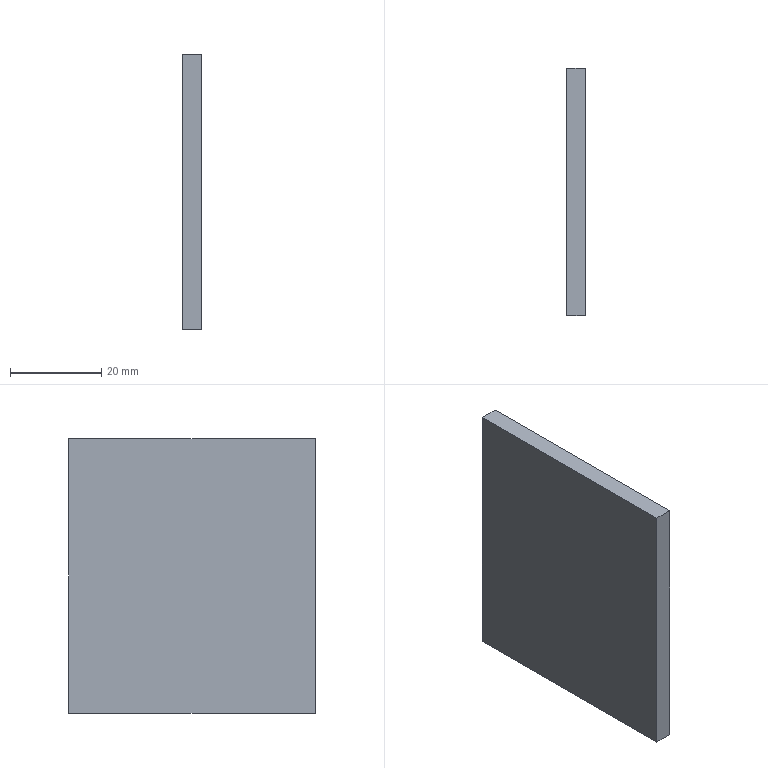Component | SolidWorks | RubberPlate-1 | 1 solid | 6 faces | box 4 x 54 x 60 mm | volume 12960 mm3 | plane 6
build123d program:
from build123d import *

# Parameters (mm, degrees)
SKETCH1_W           = 54
SKETCH1_H           = 60
BOSS_EXTRUDE1_DEPTH = 4


with BuildPart() as part:
    # Sketch1 → Boss-Extrude1 (new body)
    with BuildSketch(Plane(origin=(0, 0, -2), x_dir=(-1, 0, 0), z_dir=(0, 0, -1))):
        Rectangle(SKETCH1_W, SKETCH1_H)
    extrude(amount=-BOSS_EXTRUDE1_DEPTH)


solid = part.part

# Placed as in the assembly
solid = solid.moved(Location((-386, 405.75, -73.487), (90, -90, 0)))
STEP:
#1=COLOUR_RGB('',0.7922,0.8196,0.9333);
#2=FILL_AREA_STYLE_COLOUR('',#1);
#3=FILL_AREA_STYLE('',(#2));
#4=SURFACE_STYLE_FILL_AREA(#3);
#5=SURFACE_SIDE_STYLE('',(#4));
#6=SURFACE_STYLE_USAGE(.BOTH.,#5);
#7=PRESENTATION_STYLE_ASSIGNMENT((#6));
#8=CARTESIAN_POINT('',(-15.118,17.037,-1.712));
#9=VERTEX_POINT('',#8);
#10=CARTESIAN_POINT('',(-15.118,14.911,-1.712));
#11=VERTEX_POINT('',#10);
#12=CARTESIAN_POINT('',(-15.118,17.037,-1.712));
#13=DIRECTION('',(-0.,-1.,0.));
#14=VECTOR('',#13,39.37);
#15=LINE('',#12,#14);
#16=EDGE_CURVE('',#9,#11,#15,.T.);
#17=ORIENTED_EDGE('',*,*,#16,.F.);
#18=CARTESIAN_POINT('',(-15.276,17.037,-1.712));
#19=VERTEX_POINT('',#18);
#20=CARTESIAN_POINT('',(-15.276,17.037,-1.712));
#21=DIRECTION('',(1.,-0.,0.));
#22=VECTOR('',#21,39.37);
#23=LINE('',#20,#22);
#24=EDGE_CURVE('',#19,#9,#23,.T.);
#25=ORIENTED_EDGE('',*,*,#24,.F.);
#26=CARTESIAN_POINT('',(-15.276,14.911,-1.712));
#27=VERTEX_POINT('',#26);
#28=CARTESIAN_POINT('',(-15.276,17.037,-1.712));
#29=DIRECTION('',(-0.,-1.,0.));
#30=VECTOR('',#29,39.37);
#31=LINE('',#28,#30);
#32=EDGE_CURVE('',#19,#27,#31,.T.);
#33=ORIENTED_EDGE('',*,*,#32,.T.);
#34=CARTESIAN_POINT('',(-15.276,14.911,-1.712));
#35=DIRECTION('',(1.,-0.,0.));
#36=VECTOR('',#35,39.37);
#37=LINE('',#34,#36);
#38=EDGE_CURVE('',#27,#11,#37,.T.);
#39=ORIENTED_EDGE('',*,*,#38,.T.);
#40=EDGE_LOOP('',(#17,#25,#33,#39));
#41=FACE_OUTER_BOUND('',#40,.T.);
#42=CARTESIAN_POINT('',(-15.276,17.037,-1.712));
#43=DIRECTION('',(-0.,0.,1.));
#44=DIRECTION('',(1.,-0.,0.));
#45=AXIS2_PLACEMENT_3D('',#42,#43,#44);
#46=PLANE('',#45);
#47=ADVANCED_FACE('',(#41),#46,.T.);
#48=CARTESIAN_POINT('',(-15.118,17.037,-4.074));
#49=VERTEX_POINT('',#48);
#50=CARTESIAN_POINT('',(-15.118,17.037,-4.074));
#51=DIRECTION('',(-0.,0.,1.));
#52=VECTOR('',#51,39.37);
#53=LINE('',#50,#52);
#54=EDGE_CURVE('',#49,#9,#53,.T.);
#55=ORIENTED_EDGE('',*,*,#54,.F.);
#56=CARTESIAN_POINT('',(-15.276,17.037,-4.074));
#57=VERTEX_POINT('',#56);
#58=CARTESIAN_POINT('',(-15.276,17.037,-4.074));
#59=DIRECTION('',(1.,-0.,0.));
#60=VECTOR('',#59,39.37);
#61=LINE('',#58,#60);
#62=EDGE_CURVE('',#57,#49,#61,.T.);
#63=ORIENTED_EDGE('',*,*,#62,.F.);
#64=CARTESIAN_POINT('',(-15.276,17.037,-4.074));
#65=DIRECTION('',(-0.,0.,1.));
#66=VECTOR('',#65,39.37);
#67=LINE('',#64,#66);
#68=EDGE_CURVE('',#57,#19,#67,.T.);
#69=ORIENTED_EDGE('',*,*,#68,.T.);
#70=ORIENTED_EDGE('',*,*,#24,.T.);
#71=EDGE_LOOP('',(#55,#63,#69,#70));
#72=FACE_OUTER_BOUND('',#71,.T.);
#73=CARTESIAN_POINT('',(-15.276,17.037,-4.074));
#74=DIRECTION('',(0.,1.,-0.));
#75=DIRECTION('',(0.,-0.,-1.));
#76=AXIS2_PLACEMENT_3D('',#73,#74,#75);
#77=PLANE('',#76);
#78=ADVANCED_FACE('',(#72),#77,.T.);
#79=CARTESIAN_POINT('',(-15.118,14.911,-4.074));
#80=VERTEX_POINT('',#79);
#81=CARTESIAN_POINT('',(-15.118,14.911,-4.074));
#82=DIRECTION('',(0.,1.,-0.));
#83=VECTOR('',#82,39.37);
#84=LINE('',#81,#83);
#85=EDGE_CURVE('',#80,#49,#84,.T.);
#86=ORIENTED_EDGE('',*,*,#85,.F.);
#87=CARTESIAN_POINT('',(-15.276,14.911,-4.074));
#88=VERTEX_POINT('',#87);
#89=CARTESIAN_POINT('',(-15.276,14.911,-4.074));
#90=DIRECTION('',(1.,-0.,0.));
#91=VECTOR('',#90,39.37);
#92=LINE('',#89,#91);
#93=EDGE_CURVE('',#88,#80,#92,.T.);
#94=ORIENTED_EDGE('',*,*,#93,.F.);
#95=CARTESIAN_POINT('',(-15.276,14.911,-4.074));
#96=DIRECTION('',(0.,1.,-0.));
#97=VECTOR('',#96,39.37);
#98=LINE('',#95,#97);
#99=EDGE_CURVE('',#88,#57,#98,.T.);
#100=ORIENTED_EDGE('',*,*,#99,.T.);
#101=ORIENTED_EDGE('',*,*,#62,.T.);
#102=EDGE_LOOP('',(#86,#94,#100,#101));
#103=FACE_OUTER_BOUND('',#102,.T.);
#104=CARTESIAN_POINT('',(-15.276,14.911,-4.074));
#105=DIRECTION('',(0.,-0.,-1.));
#106=DIRECTION('',(-1.,0.,-0.));
#107=AXIS2_PLACEMENT_3D('',#104,#105,#106);
#108=PLANE('',#107);
#109=ADVANCED_FACE('',(#103),#108,.T.);
#110=CARTESIAN_POINT('',(-15.118,14.911,-1.712));
#111=DIRECTION('',(0.,-0.,-1.));
#112=VECTOR('',#111,39.37);
#113=LINE('',#110,#112);
#114=EDGE_CURVE('',#11,#80,#113,.T.);
#115=ORIENTED_EDGE('',*,*,#114,.F.);
#116=ORIENTED_EDGE('',*,*,#38,.F.);
#117=CARTESIAN_POINT('',(-15.276,14.911,-1.712));
#118=DIRECTION('',(0.,-0.,-1.));
#119=VECTOR('',#118,39.37);
#120=LINE('',#117,#119);
#121=EDGE_CURVE('',#27,#88,#120,.T.);
#122=ORIENTED_EDGE('',*,*,#121,.T.);
#123=ORIENTED_EDGE('',*,*,#93,.T.);
#124=EDGE_LOOP('',(#115,#116,#122,#123));
#125=FACE_OUTER_BOUND('',#124,.T.);
#126=CARTESIAN_POINT('',(-15.276,14.911,-1.712));
#127=DIRECTION('',(-0.,-1.,0.));
#128=DIRECTION('',(-0.,0.,1.));
#129=AXIS2_PLACEMENT_3D('',#126,#127,#128);
#130=PLANE('',#129);
#131=ADVANCED_FACE('',(#125),#130,.T.);
#132=ORIENTED_EDGE('',*,*,#32,.F.);
#133=ORIENTED_EDGE('',*,*,#68,.F.);
#134=ORIENTED_EDGE('',*,*,#99,.F.);
#135=ORIENTED_EDGE('',*,*,#121,.F.);
#136=EDGE_LOOP('',(#132,#133,#134,#135));
#137=FACE_OUTER_BOUND('',#136,.T.);
#138=CARTESIAN_POINT('',(-15.276,15.974,-2.893));
#139=DIRECTION('',(1.,-0.,0.));
#140=DIRECTION('',(-0.,-1.,0.));
#141=AXIS2_PLACEMENT_3D('',#138,#139,#140);
#142=PLANE('',#141);
#143=ADVANCED_FACE('',(#137),#142,.F.);
#144=ORIENTED_EDGE('',*,*,#16,.T.);
#145=ORIENTED_EDGE('',*,*,#114,.T.);
#146=ORIENTED_EDGE('',*,*,#85,.T.);
#147=ORIENTED_EDGE('',*,*,#54,.T.);
#148=EDGE_LOOP('',(#144,#145,#146,#147));
#149=FACE_OUTER_BOUND('',#148,.T.);
#150=CARTESIAN_POINT('',(-15.118,15.974,-2.893));
#151=DIRECTION('',(1.,-0.,0.));
#152=DIRECTION('',(-0.,-1.,0.));
#153=AXIS2_PLACEMENT_3D('',#150,#151,#152);
#154=PLANE('',#153);
#155=ADVANCED_FACE('',(#149),#154,.T.);
#156=CLOSED_SHELL('',(#47,#78,#109,#131,#143,#155));
#157=MANIFOLD_SOLID_BREP('',#156);
#158=STYLED_ITEM('',(#7),#157);
#159=(LENGTH_UNIT()NAMED_UNIT(*)SI_UNIT($,.METRE.));
#160=LENGTH_MEASURE_WITH_UNIT(LENGTH_MEASURE(0.0254),#159);
#161=DIMENSIONAL_EXPONENTS(1.,0.,0.,0.,0.,0.,0.);
#162=(CONVERSION_BASED_UNIT('',#160)LENGTH_UNIT()NAMED_UNIT(#161));
#163=UNCERTAINTY_MEASURE_WITH_UNIT(LENGTH_MEASURE(0.00001),#162,'','');
#164=(NAMED_UNIT(*)PLANE_ANGLE_UNIT()SI_UNIT($,.RADIAN.));
#165=(NAMED_UNIT(*)SI_UNIT($,.STERADIAN.)SOLID_ANGLE_UNIT());
#166=(GEOMETRIC_REPRESENTATION_CONTEXT(3)GLOBAL_UNCERTAINTY_ASSIGNED_CONTEXT((#163))GLOBAL_UNIT_ASSIGNED_CONTEXT((#162,#164,#165))REPRESENTATION_CONTEXT('',''));
#167=MECHANICAL_DESIGN_GEOMETRIC_PRESENTATION_REPRESENTATION('',(#158),#166);
#168=PRESENTATION_LAYER_ASSIGNMENT('','',(#158));
#169=CARTESIAN_POINT('',(0.,0.,0.));
#170=DIRECTION('',(0.,0.,1.));
#171=DIRECTION('',(1.,0.,0.));
#172=AXIS2_PLACEMENT_3D('',#169,#170,#171);
#173=(LENGTH_UNIT()NAMED_UNIT(*)SI_UNIT($,.METRE.));
#174=LENGTH_MEASURE_WITH_UNIT(LENGTH_MEASURE(0.0254),#173);
#175=DIMENSIONAL_EXPONENTS(1.,0.,0.,0.,0.,0.,0.);
#176=(CONVERSION_BASED_UNIT('',#174)LENGTH_UNIT()NAMED_UNIT(#175));
#177=UNCERTAINTY_MEASURE_WITH_UNIT(LENGTH_MEASURE(0.00001),#176,'','');
#178=(NAMED_UNIT(*)PLANE_ANGLE_UNIT()SI_UNIT($,.RADIAN.));
#179=(NAMED_UNIT(*)SI_UNIT($,.STERADIAN.)SOLID_ANGLE_UNIT());
#180=(GEOMETRIC_REPRESENTATION_CONTEXT(3)GLOBAL_UNCERTAINTY_ASSIGNED_CONTEXT((#177))GLOBAL_UNIT_ASSIGNED_CONTEXT((#176,#178,#179))REPRESENTATION_CONTEXT('',''));
#181=ADVANCED_BREP_SHAPE_REPRESENTATION('',(#157,#172),#180);